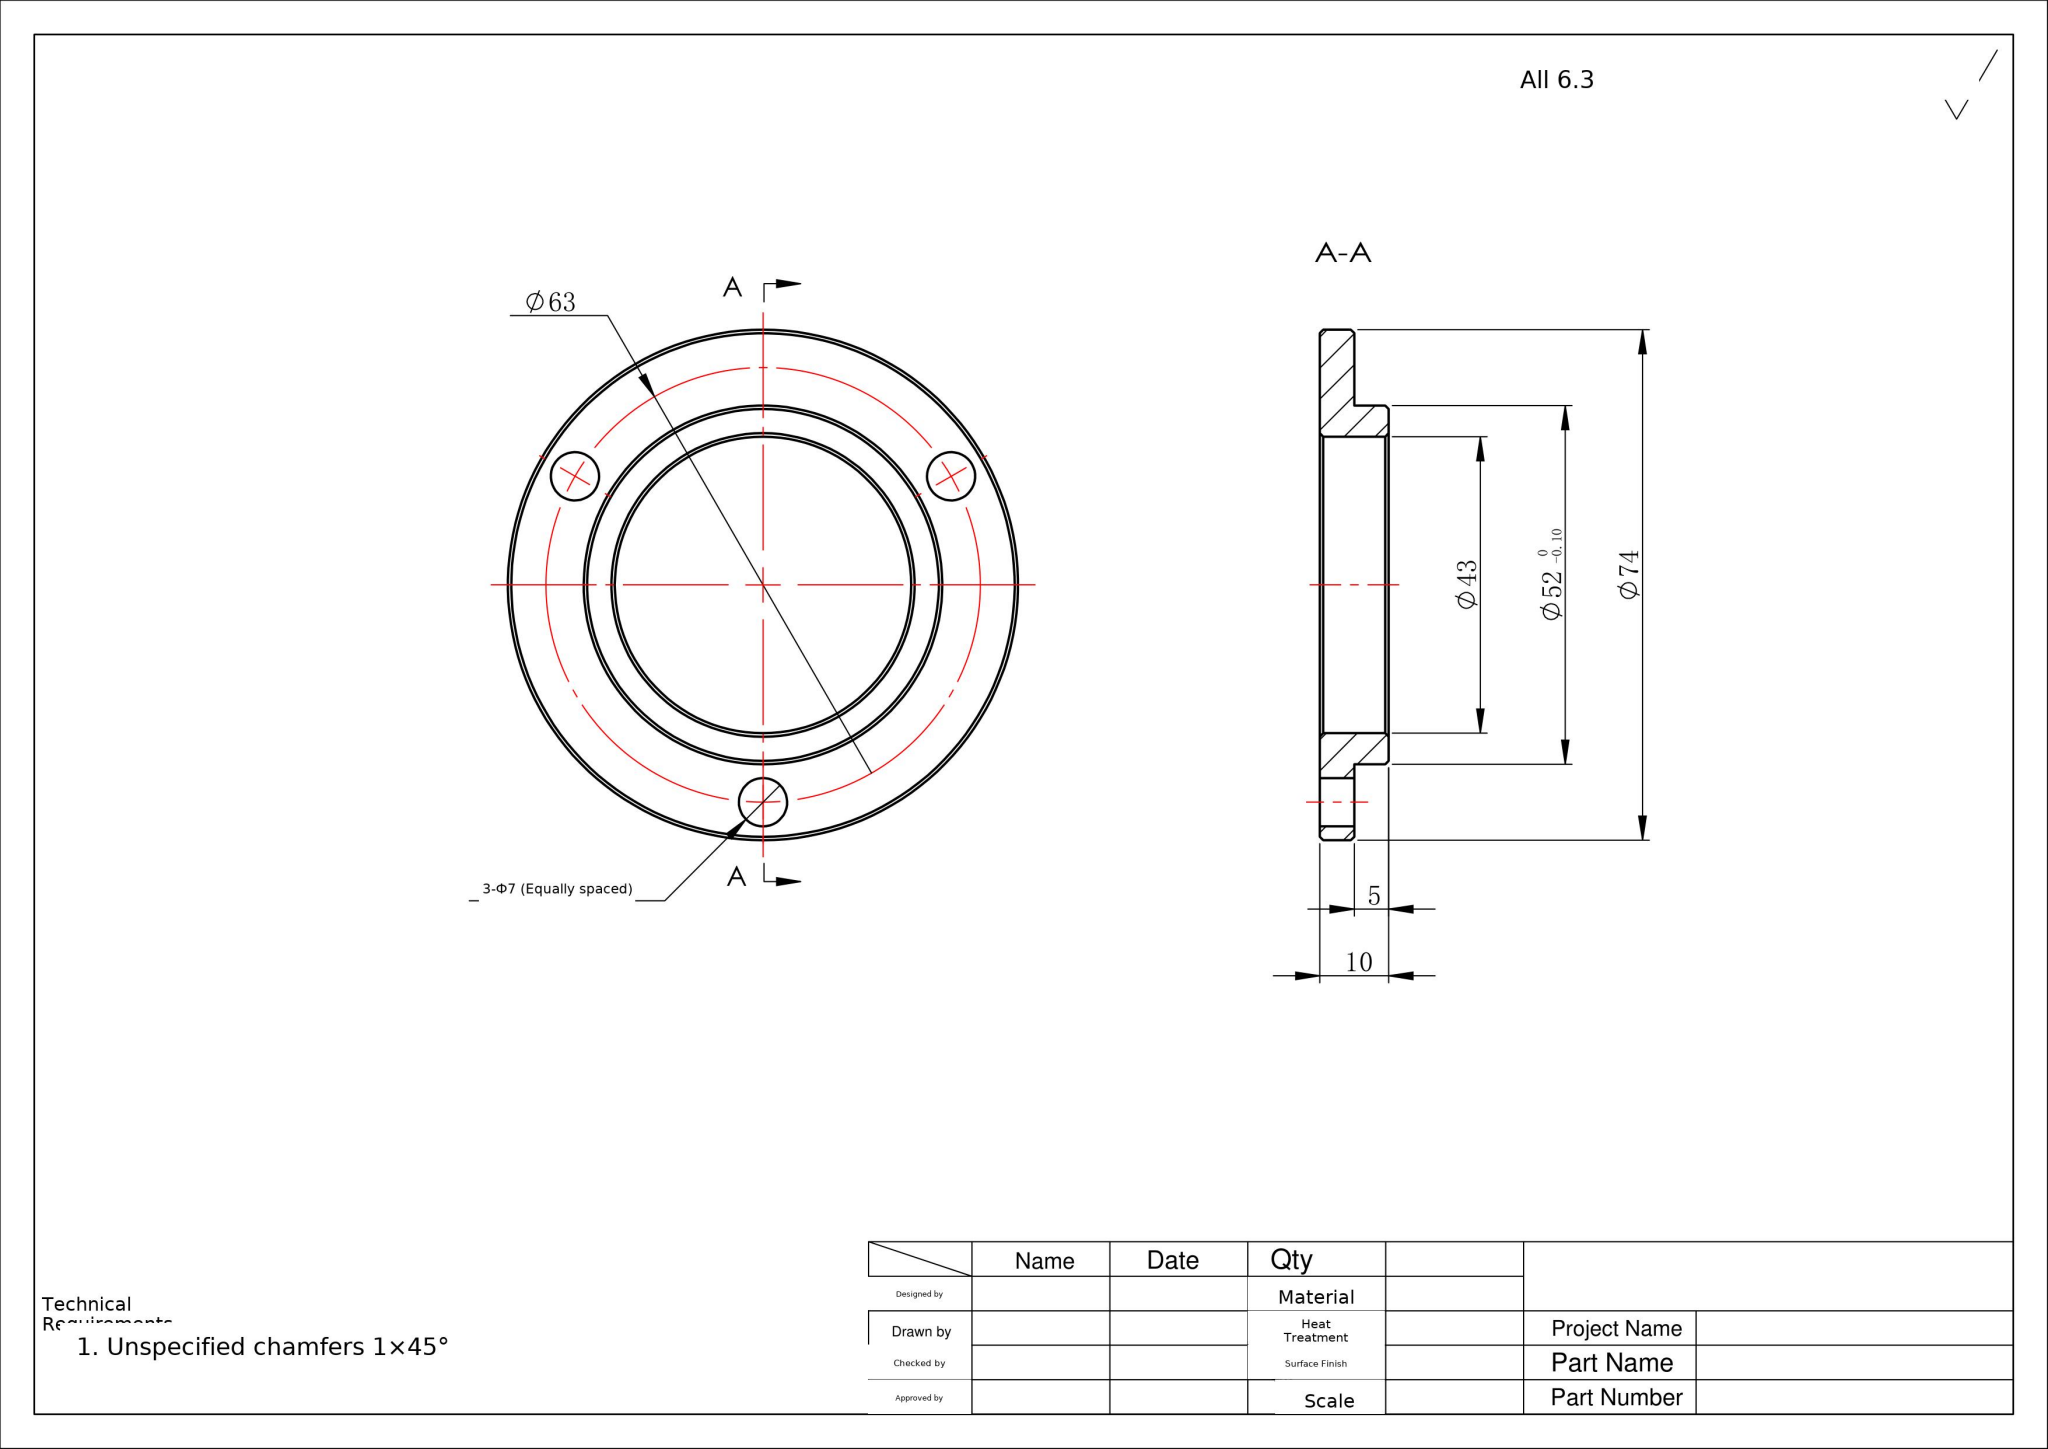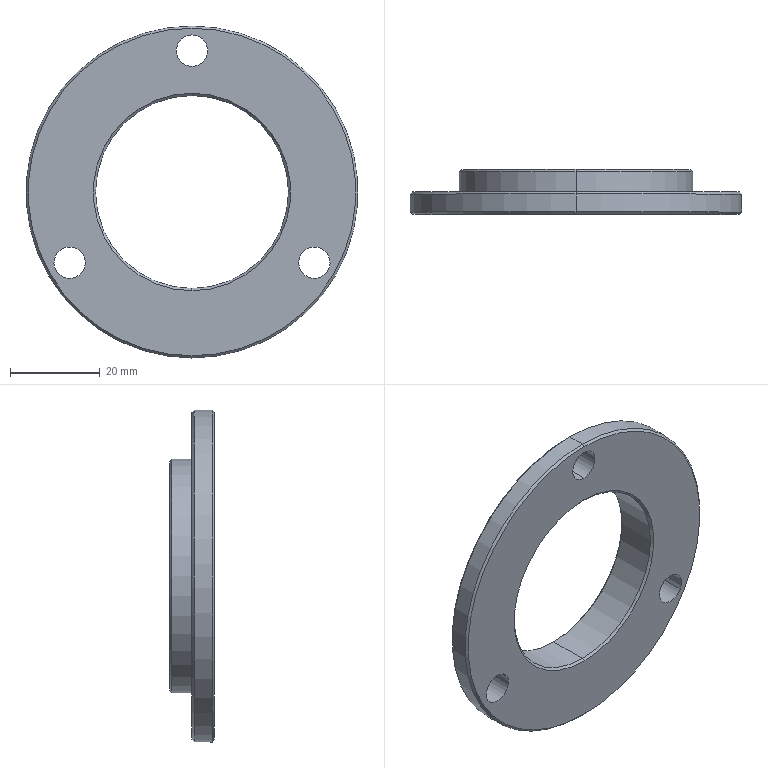Part | SolidWorks | mm | 1 solid | 25 faces | box 74 x 10 x 74 mm | volume 16911 mm3 | cylinder 12 | cone 10 | plane 3 | commonest cylinder face diameters 7 x6 43 x2 52 x2 74 x2
build123d program:
from build123d import *

# Parameters (mm, degrees)
SKETCH2_R          = 3.5
CUT_EXTRUDE1_DEPTH = 54.273
CIRPATTERN1_COUNT  = 3
CHAMFER1_SIZE      = 0.5


with BuildPart() as part:
    # Sketch1 → Revolve1 (revolve)
    with BuildSketch(Plane.XY, mode=Mode.PRIVATE) as revolve1_sk:
        Polygon((21.5, 0), (37, 0), (37, 5), (26, 5), (26, 10), (21.5, 10), align=None)
    revolve(revolve1_sk.sketch.rotate(Axis((0, 0, 0), (0, 1, 0)), 90), axis=Axis((0, 0, 0), (0, 1, 0)))

    # Sketch2 → Cut-Extrude1 (cut, through all)
    with BuildSketch(Plane.XZ):
        with Locations(Location((0, 31.5, 0), (0, 0, 270))):
            Circle(SKETCH2_R)
    cut_extrude1 = extrude(amount=-CUT_EXTRUDE1_DEPTH, mode=Mode.SUBTRACT)

    # CirPattern1: Cut-Extrude1 ×3 about axis
    cirpattern1_axis = Axis((0, 0, 0), (0, 1, 0))
    for i in range(1, CIRPATTERN1_COUNT):
        add(cut_extrude1.rotate(cirpattern1_axis, i * 360 / CIRPATTERN1_COUNT), mode=Mode.SUBTRACT)

    # Chamfer1
    chamfer1_edges = [part.edges().sort_by_distance(p)[0] for p in [
        (0, 0, 37),
        (0, 0, 21.5),
        (0, 10, 21.5),
        (0, 10, 26),
        (0, 5, 37),
    ]]
    chamfer(chamfer1_edges, length=CHAMFER1_SIZE)


solid = part.part
STEP:
#1=CARTESIAN_POINT('',(0.,5.,36.5));
#2=VERTEX_POINT('',#1);
#3=CARTESIAN_POINT('',(-0.,5.,-36.5));
#4=VERTEX_POINT('',#3);
#5=CARTESIAN_POINT('',(0.,5.,-0.));
#6=DIRECTION('',(-0.,1.,0.));
#7=DIRECTION('',(0.,0.,1.));
#8=AXIS2_PLACEMENT_3D('',#5,#6,#7);
#9=CIRCLE('',#8,36.5);
#10=EDGE_CURVE('',#2,#4,#9,.T.);
#11=ORIENTED_EDGE('',*,*,#10,.F.);
#12=CARTESIAN_POINT('',(0.,4.5,37.));
#13=VERTEX_POINT('',#12);
#14=CARTESIAN_POINT('',(0.,4.5,37.));
#15=DIRECTION('',(0.,-0.7071,0.7071));
#16=VECTOR('',#15,1000.);
#17=LINE('',#14,#16);
#18=EDGE_CURVE('',#2,#13,#17,.T.);
#19=ORIENTED_EDGE('',*,*,#18,.T.);
#20=CARTESIAN_POINT('',(-0.,4.5,-37.));
#21=VERTEX_POINT('',#20);
#22=CARTESIAN_POINT('',(0.,4.5,-0.));
#23=DIRECTION('',(0.,-1.,-0.));
#24=DIRECTION('',(0.,0.,1.));
#25=AXIS2_PLACEMENT_3D('',#22,#23,#24);
#26=CIRCLE('',#25,37.);
#27=EDGE_CURVE('',#21,#13,#26,.T.);
#28=ORIENTED_EDGE('',*,*,#27,.F.);
#29=CARTESIAN_POINT('',(-0.,4.5,-37.));
#30=DIRECTION('',(-0.,-0.7071,-0.7071));
#31=VECTOR('',#30,1000.);
#32=LINE('',#29,#31);
#33=EDGE_CURVE('',#4,#21,#32,.T.);
#34=ORIENTED_EDGE('',*,*,#33,.F.);
#35=EDGE_LOOP('',(#11,#19,#28,#34));
#36=FACE_OUTER_BOUND('',#35,.T.);
#37=CARTESIAN_POINT('',(0.,4.5,-0.));
#38=DIRECTION('',(0.,-1.,-0.));
#39=DIRECTION('',(-0.,0.,-1.));
#40=AXIS2_PLACEMENT_3D('',#37,#38,#39);
#41=CONICAL_SURFACE('',#40,37.,0.7854);
#42=ADVANCED_FACE('',(#36),#41,.T.);
#43=CARTESIAN_POINT('',(0.,0.,-36.5));
#44=VERTEX_POINT('',#43);
#45=CARTESIAN_POINT('',(0.,-0.,36.5));
#46=VERTEX_POINT('',#45);
#47=CARTESIAN_POINT('',(0.,0.,-0.));
#48=DIRECTION('',(0.,-1.,-0.));
#49=DIRECTION('',(-0.,-0.,-1.));
#50=AXIS2_PLACEMENT_3D('',#47,#48,#49);
#51=CIRCLE('',#50,36.5);
#52=EDGE_CURVE('',#44,#46,#51,.T.);
#53=ORIENTED_EDGE('',*,*,#52,.F.);
#54=CARTESIAN_POINT('',(-0.,0.5,-37.));
#55=VERTEX_POINT('',#54);
#56=CARTESIAN_POINT('',(0.,-0.,-36.5));
#57=DIRECTION('',(0.,0.7071,-0.7071));
#58=VECTOR('',#57,1000.);
#59=LINE('',#56,#58);
#60=EDGE_CURVE('',#44,#55,#59,.T.);
#61=ORIENTED_EDGE('',*,*,#60,.T.);
#62=CARTESIAN_POINT('',(0.,0.5,37.));
#63=VERTEX_POINT('',#62);
#64=CARTESIAN_POINT('',(0.,0.5,-0.));
#65=DIRECTION('',(-0.,1.,0.));
#66=DIRECTION('',(-0.,0.,-1.));
#67=AXIS2_PLACEMENT_3D('',#64,#65,#66);
#68=CIRCLE('',#67,37.);
#69=EDGE_CURVE('',#63,#55,#68,.T.);
#70=ORIENTED_EDGE('',*,*,#69,.F.);
#71=CARTESIAN_POINT('',(0.,0.,36.5));
#72=DIRECTION('',(0.,0.7071,0.7071));
#73=VECTOR('',#72,1000.);
#74=LINE('',#71,#73);
#75=EDGE_CURVE('',#46,#63,#74,.T.);
#76=ORIENTED_EDGE('',*,*,#75,.F.);
#77=EDGE_LOOP('',(#53,#61,#70,#76));
#78=FACE_OUTER_BOUND('',#77,.T.);
#79=CARTESIAN_POINT('',(0.,0.,-0.));
#80=DIRECTION('',(-0.,1.,0.));
#81=DIRECTION('',(0.,0.,1.));
#82=AXIS2_PLACEMENT_3D('',#79,#80,#81);
#83=CONICAL_SURFACE('',#82,36.5,0.7854);
#84=ADVANCED_FACE('',(#78),#83,.T.);
#85=CARTESIAN_POINT('',(0.,0.5,21.5));
#86=VERTEX_POINT('',#85);
#87=CARTESIAN_POINT('',(-0.,0.5,-21.5));
#88=VERTEX_POINT('',#87);
#89=CARTESIAN_POINT('',(0.,0.5,-0.));
#90=DIRECTION('',(0.,-1.,-0.));
#91=DIRECTION('',(-0.,0.,-1.));
#92=AXIS2_PLACEMENT_3D('',#89,#90,#91);
#93=CIRCLE('',#92,21.5);
#94=EDGE_CURVE('',#86,#88,#93,.T.);
#95=ORIENTED_EDGE('',*,*,#94,.F.);
#96=CARTESIAN_POINT('',(0.,0.,22.));
#97=VERTEX_POINT('',#96);
#98=CARTESIAN_POINT('',(0.,0.5,21.5));
#99=DIRECTION('',(0.,-0.7071,0.7071));
#100=VECTOR('',#99,1000.);
#101=LINE('',#98,#100);
#102=EDGE_CURVE('',#86,#97,#101,.T.);
#103=ORIENTED_EDGE('',*,*,#102,.T.);
#104=CARTESIAN_POINT('',(-0.,0.,-22.));
#105=VERTEX_POINT('',#104);
#106=CARTESIAN_POINT('',(0.,0.,-0.));
#107=DIRECTION('',(-0.,1.,0.));
#108=DIRECTION('',(-0.,-0.,-1.));
#109=AXIS2_PLACEMENT_3D('',#106,#107,#108);
#110=CIRCLE('',#109,22.);
#111=EDGE_CURVE('',#105,#97,#110,.T.);
#112=ORIENTED_EDGE('',*,*,#111,.F.);
#113=CARTESIAN_POINT('',(-0.,0.5,-21.5));
#114=DIRECTION('',(-0.,-0.7071,-0.7071));
#115=VECTOR('',#114,1000.);
#116=LINE('',#113,#115);
#117=EDGE_CURVE('',#88,#105,#116,.T.);
#118=ORIENTED_EDGE('',*,*,#117,.F.);
#119=EDGE_LOOP('',(#95,#103,#112,#118));
#120=FACE_OUTER_BOUND('',#119,.T.);
#121=CARTESIAN_POINT('',(0.,0.5,-0.));
#122=DIRECTION('',(0.,-1.,-0.));
#123=DIRECTION('',(-0.,0.,-1.));
#124=AXIS2_PLACEMENT_3D('',#121,#122,#123);
#125=CONICAL_SURFACE('',#124,21.5,0.7854);
#126=ADVANCED_FACE('',(#120),#125,.F.);
#127=CARTESIAN_POINT('',(0.,10.,25.5));
#128=VERTEX_POINT('',#127);
#129=CARTESIAN_POINT('',(-0.,10.,-25.5));
#130=VERTEX_POINT('',#129);
#131=CARTESIAN_POINT('',(0.,10.,-0.));
#132=DIRECTION('',(-0.,1.,0.));
#133=DIRECTION('',(0.,0.,1.));
#134=AXIS2_PLACEMENT_3D('',#131,#132,#133);
#135=CIRCLE('',#134,25.5);
#136=EDGE_CURVE('',#128,#130,#135,.T.);
#137=ORIENTED_EDGE('',*,*,#136,.F.);
#138=CARTESIAN_POINT('',(0.,9.5,26.));
#139=VERTEX_POINT('',#138);
#140=CARTESIAN_POINT('',(0.,9.5,26.));
#141=DIRECTION('',(0.,-0.7071,0.7071));
#142=VECTOR('',#141,1000.);
#143=LINE('',#140,#142);
#144=EDGE_CURVE('',#128,#139,#143,.T.);
#145=ORIENTED_EDGE('',*,*,#144,.T.);
#146=CARTESIAN_POINT('',(-0.,9.5,-26.));
#147=VERTEX_POINT('',#146);
#148=CARTESIAN_POINT('',(0.,9.5,-0.));
#149=DIRECTION('',(0.,-1.,-0.));
#150=DIRECTION('',(0.,0.,1.));
#151=AXIS2_PLACEMENT_3D('',#148,#149,#150);
#152=CIRCLE('',#151,26.);
#153=EDGE_CURVE('',#147,#139,#152,.T.);
#154=ORIENTED_EDGE('',*,*,#153,.F.);
#155=CARTESIAN_POINT('',(-0.,9.5,-26.));
#156=DIRECTION('',(-0.,-0.7071,-0.7071));
#157=VECTOR('',#156,1000.);
#158=LINE('',#155,#157);
#159=EDGE_CURVE('',#130,#147,#158,.T.);
#160=ORIENTED_EDGE('',*,*,#159,.F.);
#161=EDGE_LOOP('',(#137,#145,#154,#160));
#162=FACE_OUTER_BOUND('',#161,.T.);
#163=CARTESIAN_POINT('',(0.,9.5,-0.));
#164=DIRECTION('',(0.,-1.,-0.));
#165=DIRECTION('',(-0.,0.,-1.));
#166=AXIS2_PLACEMENT_3D('',#163,#164,#165);
#167=CONICAL_SURFACE('',#166,26.,0.7854);
#168=ADVANCED_FACE('',(#162),#167,.T.);
#169=CARTESIAN_POINT('',(-0.,9.5,-21.5));
#170=VERTEX_POINT('',#169);
#171=CARTESIAN_POINT('',(0.,9.5,21.5));
#172=VERTEX_POINT('',#171);
#173=CARTESIAN_POINT('',(0.,9.5,-0.));
#174=DIRECTION('',(-0.,1.,0.));
#175=DIRECTION('',(0.,0.,1.));
#176=AXIS2_PLACEMENT_3D('',#173,#174,#175);
#177=CIRCLE('',#176,21.5);
#178=EDGE_CURVE('',#170,#172,#177,.T.);
#179=ORIENTED_EDGE('',*,*,#178,.F.);
#180=CARTESIAN_POINT('',(0.,10.,-22.));
#181=VERTEX_POINT('',#180);
#182=CARTESIAN_POINT('',(0.,10.,-22.));
#183=DIRECTION('',(0.,0.7071,-0.7071));
#184=VECTOR('',#183,1000.);
#185=LINE('',#182,#184);
#186=EDGE_CURVE('',#170,#181,#185,.T.);
#187=ORIENTED_EDGE('',*,*,#186,.T.);
#188=CARTESIAN_POINT('',(0.,10.,22.));
#189=VERTEX_POINT('',#188);
#190=CARTESIAN_POINT('',(0.,10.,-0.));
#191=DIRECTION('',(0.,-1.,-0.));
#192=DIRECTION('',(0.,0.,1.));
#193=AXIS2_PLACEMENT_3D('',#190,#191,#192);
#194=CIRCLE('',#193,22.);
#195=EDGE_CURVE('',#189,#181,#194,.T.);
#196=ORIENTED_EDGE('',*,*,#195,.F.);
#197=CARTESIAN_POINT('',(0.,10.,22.));
#198=DIRECTION('',(0.,0.7071,0.7071));
#199=VECTOR('',#198,1000.);
#200=LINE('',#197,#199);
#201=EDGE_CURVE('',#172,#189,#200,.T.);
#202=ORIENTED_EDGE('',*,*,#201,.F.);
#203=EDGE_LOOP('',(#179,#187,#196,#202));
#204=FACE_OUTER_BOUND('',#203,.T.);
#205=CARTESIAN_POINT('',(0.,10.,-0.));
#206=DIRECTION('',(-0.,1.,0.));
#207=DIRECTION('',(0.,0.,1.));
#208=AXIS2_PLACEMENT_3D('',#205,#206,#207);
#209=CONICAL_SURFACE('',#208,22.,0.7854);
#210=ADVANCED_FACE('',(#204),#209,.F.);
#211=CARTESIAN_POINT('',(-24.249,5.,-14.));
#212=VERTEX_POINT('',#211);
#213=CARTESIAN_POINT('',(-30.311,5.,-17.5));
#214=VERTEX_POINT('',#213);
#215=CARTESIAN_POINT('',(-27.28,5.,-15.75));
#216=DIRECTION('',(-0.,1.,0.));
#217=DIRECTION('',(-0.866,0.,-0.5));
#218=AXIS2_PLACEMENT_3D('',#215,#216,#217);
#219=CIRCLE('',#218,3.5);
#220=EDGE_CURVE('',#212,#214,#219,.T.);
#221=ORIENTED_EDGE('',*,*,#220,.T.);
#222=CARTESIAN_POINT('',(-30.311,0.,-17.5));
#223=VERTEX_POINT('',#222);
#224=CARTESIAN_POINT('',(-30.311,10.,-17.5));
#225=DIRECTION('',(0.,-1.,-0.));
#226=VECTOR('',#225,1000.);
#227=LINE('',#224,#226);
#228=EDGE_CURVE('',#214,#223,#227,.T.);
#229=ORIENTED_EDGE('',*,*,#228,.T.);
#230=CARTESIAN_POINT('',(-24.249,0.,-14.));
#231=VERTEX_POINT('',#230);
#232=CARTESIAN_POINT('',(-27.28,0.,-15.75));
#233=DIRECTION('',(0.,-1.,-0.));
#234=DIRECTION('',(0.866,0.,0.5));
#235=AXIS2_PLACEMENT_3D('',#232,#233,#234);
#236=CIRCLE('',#235,3.5);
#237=EDGE_CURVE('',#223,#231,#236,.T.);
#238=ORIENTED_EDGE('',*,*,#237,.T.);
#239=CARTESIAN_POINT('',(-24.249,10.,-14.));
#240=DIRECTION('',(0.,-1.,-0.));
#241=VECTOR('',#240,1000.);
#242=LINE('',#239,#241);
#243=EDGE_CURVE('',#212,#231,#242,.T.);
#244=ORIENTED_EDGE('',*,*,#243,.F.);
#245=EDGE_LOOP('',(#221,#229,#238,#244));
#246=FACE_OUTER_BOUND('',#245,.T.);
#247=CARTESIAN_POINT('',(-27.28,10.,-15.75));
#248=DIRECTION('',(0.,-1.,-0.));
#249=DIRECTION('',(0.866,0.,0.5));
#250=AXIS2_PLACEMENT_3D('',#247,#248,#249);
#251=CYLINDRICAL_SURFACE('',#250,3.5);
#252=ADVANCED_FACE('',(#246),#251,.F.);
#253=CARTESIAN_POINT('',(24.249,5.,-14.));
#254=VERTEX_POINT('',#253);
#255=CARTESIAN_POINT('',(30.311,5.,-17.5));
#256=VERTEX_POINT('',#255);
#257=CARTESIAN_POINT('',(27.28,5.,-15.75));
#258=DIRECTION('',(-0.,1.,0.));
#259=DIRECTION('',(0.866,0.,-0.5));
#260=AXIS2_PLACEMENT_3D('',#257,#258,#259);
#261=CIRCLE('',#260,3.5);
#262=EDGE_CURVE('',#254,#256,#261,.T.);
#263=ORIENTED_EDGE('',*,*,#262,.T.);
#264=CARTESIAN_POINT('',(30.311,0.,-17.5));
#265=VERTEX_POINT('',#264);
#266=CARTESIAN_POINT('',(30.311,10.,-17.5));
#267=DIRECTION('',(0.,-1.,-0.));
#268=VECTOR('',#267,1000.);
#269=LINE('',#266,#268);
#270=EDGE_CURVE('',#256,#265,#269,.T.);
#271=ORIENTED_EDGE('',*,*,#270,.T.);
#272=CARTESIAN_POINT('',(24.249,0.,-14.));
#273=VERTEX_POINT('',#272);
#274=CARTESIAN_POINT('',(27.28,0.,-15.75));
#275=DIRECTION('',(0.,-1.,-0.));
#276=DIRECTION('',(-0.866,0.,0.5));
#277=AXIS2_PLACEMENT_3D('',#274,#275,#276);
#278=CIRCLE('',#277,3.5);
#279=EDGE_CURVE('',#265,#273,#278,.T.);
#280=ORIENTED_EDGE('',*,*,#279,.T.);
#281=CARTESIAN_POINT('',(24.249,10.,-14.));
#282=DIRECTION('',(0.,-1.,-0.));
#283=VECTOR('',#282,1000.);
#284=LINE('',#281,#283);
#285=EDGE_CURVE('',#254,#273,#284,.T.);
#286=ORIENTED_EDGE('',*,*,#285,.F.);
#287=EDGE_LOOP('',(#263,#271,#280,#286));
#288=FACE_OUTER_BOUND('',#287,.T.);
#289=CARTESIAN_POINT('',(27.28,10.,-15.75));
#290=DIRECTION('',(0.,-1.,-0.));
#291=DIRECTION('',(-0.866,0.,0.5));
#292=AXIS2_PLACEMENT_3D('',#289,#290,#291);
#293=CYLINDRICAL_SURFACE('',#292,3.5);
#294=ADVANCED_FACE('',(#288),#293,.F.);
#295=CARTESIAN_POINT('',(-0.,5.,28.));
#296=VERTEX_POINT('',#295);
#297=CARTESIAN_POINT('',(-0.,5.,35.));
#298=VERTEX_POINT('',#297);
#299=CARTESIAN_POINT('',(-0.,5.,31.5));
#300=DIRECTION('',(-0.,1.,0.));
#301=DIRECTION('',(0.,0.,1.));
#302=AXIS2_PLACEMENT_3D('',#299,#300,#301);
#303=CIRCLE('',#302,3.5);
#304=EDGE_CURVE('',#296,#298,#303,.T.);
#305=ORIENTED_EDGE('',*,*,#304,.T.);
#306=CARTESIAN_POINT('',(-0.,-0.,35.));
#307=VERTEX_POINT('',#306);
#308=CARTESIAN_POINT('',(-0.,10.,35.));
#309=DIRECTION('',(0.,-1.,-0.));
#310=VECTOR('',#309,1000.);
#311=LINE('',#308,#310);
#312=EDGE_CURVE('',#298,#307,#311,.T.);
#313=ORIENTED_EDGE('',*,*,#312,.T.);
#314=CARTESIAN_POINT('',(-0.,-0.,28.));
#315=VERTEX_POINT('',#314);
#316=CARTESIAN_POINT('',(-0.,-0.,31.5));
#317=DIRECTION('',(0.,-1.,-0.));
#318=DIRECTION('',(-0.,0.,-1.));
#319=AXIS2_PLACEMENT_3D('',#316,#317,#318);
#320=CIRCLE('',#319,3.5);
#321=EDGE_CURVE('',#307,#315,#320,.T.);
#322=ORIENTED_EDGE('',*,*,#321,.T.);
#323=CARTESIAN_POINT('',(-0.,10.,28.));
#324=DIRECTION('',(0.,-1.,-0.));
#325=VECTOR('',#324,1000.);
#326=LINE('',#323,#325);
#327=EDGE_CURVE('',#296,#315,#326,.T.);
#328=ORIENTED_EDGE('',*,*,#327,.F.);
#329=EDGE_LOOP('',(#305,#313,#322,#328));
#330=FACE_OUTER_BOUND('',#329,.T.);
#331=CARTESIAN_POINT('',(-0.,10.,31.5));
#332=DIRECTION('',(0.,-1.,-0.));
#333=DIRECTION('',(-0.,0.,-1.));
#334=AXIS2_PLACEMENT_3D('',#331,#332,#333);
#335=CYLINDRICAL_SURFACE('',#334,3.5);
#336=ADVANCED_FACE('',(#330),#335,.F.);
#337=ORIENTED_EDGE('',*,*,#178,.T.);
#338=CARTESIAN_POINT('',(0.,0.,21.5));
#339=DIRECTION('',(0.,-1.,-0.));
#340=VECTOR('',#339,1000.);
#341=LINE('',#338,#340);
#342=EDGE_CURVE('',#172,#86,#341,.T.);
#343=ORIENTED_EDGE('',*,*,#342,.T.);
#344=ORIENTED_EDGE('',*,*,#94,.T.);
#345=CARTESIAN_POINT('',(-0.,-0.,-21.5));
#346=DIRECTION('',(0.,-1.,-0.));
#347=VECTOR('',#346,1000.);
#348=LINE('',#345,#347);
#349=EDGE_CURVE('',#170,#88,#348,.T.);
#350=ORIENTED_EDGE('',*,*,#349,.F.);
#351=EDGE_LOOP('',(#337,#343,#344,#350));
#352=FACE_OUTER_BOUND('',#351,.T.);
#353=CARTESIAN_POINT('',(0.,0.,-0.));
#354=DIRECTION('',(0.,-1.,-0.));
#355=DIRECTION('',(-0.,-0.,-1.));
#356=AXIS2_PLACEMENT_3D('',#353,#354,#355);
#357=CYLINDRICAL_SURFACE('',#356,21.5);
#358=ADVANCED_FACE('',(#352),#357,.F.);
#359=ORIENTED_EDGE('',*,*,#153,.T.);
#360=CARTESIAN_POINT('',(0.,5.,26.));
#361=VERTEX_POINT('',#360);
#362=CARTESIAN_POINT('',(0.,0.,26.));
#363=DIRECTION('',(0.,-1.,-0.));
#364=VECTOR('',#363,1000.);
#365=LINE('',#362,#364);
#366=EDGE_CURVE('',#139,#361,#365,.T.);
#367=ORIENTED_EDGE('',*,*,#366,.T.);
#368=CARTESIAN_POINT('',(-0.,5.,-26.));
#369=VERTEX_POINT('',#368);
#370=CARTESIAN_POINT('',(0.,5.,-0.));
#371=DIRECTION('',(0.,-1.,-0.));
#372=DIRECTION('',(-0.,0.,-1.));
#373=AXIS2_PLACEMENT_3D('',#370,#371,#372);
#374=CIRCLE('',#373,26.);
#375=EDGE_CURVE('',#369,#361,#374,.T.);
#376=ORIENTED_EDGE('',*,*,#375,.F.);
#377=CARTESIAN_POINT('',(-0.,-0.,-26.));
#378=DIRECTION('',(0.,-1.,-0.));
#379=VECTOR('',#378,1000.);
#380=LINE('',#377,#379);
#381=EDGE_CURVE('',#147,#369,#380,.T.);
#382=ORIENTED_EDGE('',*,*,#381,.F.);
#383=EDGE_LOOP('',(#359,#367,#376,#382));
#384=FACE_OUTER_BOUND('',#383,.T.);
#385=CARTESIAN_POINT('',(0.,0.,-0.));
#386=DIRECTION('',(0.,-1.,-0.));
#387=DIRECTION('',(-0.,-0.,-1.));
#388=AXIS2_PLACEMENT_3D('',#385,#386,#387);
#389=CYLINDRICAL_SURFACE('',#388,26.);
#390=ADVANCED_FACE('',(#384),#389,.T.);
#391=ORIENTED_EDGE('',*,*,#27,.T.);
#392=CARTESIAN_POINT('',(0.,0.,37.));
#393=DIRECTION('',(0.,-1.,-0.));
#394=VECTOR('',#393,1000.);
#395=LINE('',#392,#394);
#396=EDGE_CURVE('',#13,#63,#395,.T.);
#397=ORIENTED_EDGE('',*,*,#396,.T.);
#398=ORIENTED_EDGE('',*,*,#69,.T.);
#399=CARTESIAN_POINT('',(-0.,-0.,-37.));
#400=DIRECTION('',(0.,-1.,-0.));
#401=VECTOR('',#400,1000.);
#402=LINE('',#399,#401);
#403=EDGE_CURVE('',#21,#55,#402,.T.);
#404=ORIENTED_EDGE('',*,*,#403,.F.);
#405=EDGE_LOOP('',(#391,#397,#398,#404));
#406=FACE_OUTER_BOUND('',#405,.T.);
#407=CARTESIAN_POINT('',(0.,0.,-0.));
#408=DIRECTION('',(0.,-1.,-0.));
#409=DIRECTION('',(-0.,-0.,-1.));
#410=AXIS2_PLACEMENT_3D('',#407,#408,#409);
#411=CYLINDRICAL_SURFACE('',#410,37.);
#412=ADVANCED_FACE('',(#406),#411,.T.);
#413=ORIENTED_EDGE('',*,*,#396,.F.);
#414=CARTESIAN_POINT('',(0.,4.5,-0.));
#415=DIRECTION('',(0.,-1.,-0.));
#416=DIRECTION('',(0.,0.,1.));
#417=AXIS2_PLACEMENT_3D('',#414,#415,#416);
#418=CIRCLE('',#417,37.);
#419=EDGE_CURVE('',#13,#21,#418,.T.);
#420=ORIENTED_EDGE('',*,*,#419,.T.);
#421=ORIENTED_EDGE('',*,*,#403,.T.);
#422=CARTESIAN_POINT('',(0.,0.5,-0.));
#423=DIRECTION('',(-0.,1.,0.));
#424=DIRECTION('',(-0.,0.,-1.));
#425=AXIS2_PLACEMENT_3D('',#422,#423,#424);
#426=CIRCLE('',#425,37.);
#427=EDGE_CURVE('',#55,#63,#426,.T.);
#428=ORIENTED_EDGE('',*,*,#427,.T.);
#429=EDGE_LOOP('',(#413,#420,#421,#428));
#430=FACE_OUTER_BOUND('',#429,.T.);
#431=CARTESIAN_POINT('',(0.,0.,-0.));
#432=DIRECTION('',(0.,-1.,-0.));
#433=DIRECTION('',(-0.,-0.,-1.));
#434=AXIS2_PLACEMENT_3D('',#431,#432,#433);
#435=CYLINDRICAL_SURFACE('',#434,37.);
#436=ADVANCED_FACE('',(#430),#435,.T.);
#437=CARTESIAN_POINT('',(0.,5.,-0.));
#438=DIRECTION('',(-0.,1.,0.));
#439=DIRECTION('',(0.,0.,1.));
#440=AXIS2_PLACEMENT_3D('',#437,#438,#439);
#441=CIRCLE('',#440,36.5);
#442=EDGE_CURVE('',#4,#2,#441,.T.);
#443=ORIENTED_EDGE('',*,*,#442,.T.);
#444=ORIENTED_EDGE('',*,*,#10,.T.);
#445=EDGE_LOOP('',(#443,#444));
#446=FACE_OUTER_BOUND('',#445,.T.);
#447=ORIENTED_EDGE('',*,*,#220,.F.);
#448=CARTESIAN_POINT('',(-27.28,5.,-15.75));
#449=DIRECTION('',(-0.,1.,0.));
#450=DIRECTION('',(-0.866,0.,-0.5));
#451=AXIS2_PLACEMENT_3D('',#448,#449,#450);
#452=CIRCLE('',#451,3.5);
#453=EDGE_CURVE('',#214,#212,#452,.T.);
#454=ORIENTED_EDGE('',*,*,#453,.F.);
#455=EDGE_LOOP('',(#447,#454));
#456=FACE_BOUND('',#455,.T.);
#457=ORIENTED_EDGE('',*,*,#262,.F.);
#458=CARTESIAN_POINT('',(27.28,5.,-15.75));
#459=DIRECTION('',(-0.,1.,0.));
#460=DIRECTION('',(0.866,0.,-0.5));
#461=AXIS2_PLACEMENT_3D('',#458,#459,#460);
#462=CIRCLE('',#461,3.5);
#463=EDGE_CURVE('',#256,#254,#462,.T.);
#464=ORIENTED_EDGE('',*,*,#463,.F.);
#465=EDGE_LOOP('',(#457,#464));
#466=FACE_BOUND('',#465,.T.);
#467=ORIENTED_EDGE('',*,*,#304,.F.);
#468=CARTESIAN_POINT('',(-0.,5.,31.5));
#469=DIRECTION('',(-0.,1.,0.));
#470=DIRECTION('',(0.,0.,1.));
#471=AXIS2_PLACEMENT_3D('',#468,#469,#470);
#472=CIRCLE('',#471,3.5);
#473=EDGE_CURVE('',#298,#296,#472,.T.);
#474=ORIENTED_EDGE('',*,*,#473,.F.);
#475=EDGE_LOOP('',(#467,#474));
#476=FACE_BOUND('',#475,.T.);
#477=ORIENTED_EDGE('',*,*,#375,.T.);
#478=CARTESIAN_POINT('',(0.,5.,-0.));
#479=DIRECTION('',(0.,-1.,-0.));
#480=DIRECTION('',(-0.,0.,-1.));
#481=AXIS2_PLACEMENT_3D('',#478,#479,#480);
#482=CIRCLE('',#481,26.);
#483=EDGE_CURVE('',#361,#369,#482,.T.);
#484=ORIENTED_EDGE('',*,*,#483,.T.);
#485=EDGE_LOOP('',(#477,#484));
#486=FACE_BOUND('',#485,.T.);
#487=CARTESIAN_POINT('',(37.,5.,0.));
#488=DIRECTION('',(-0.,1.,-0.));
#489=DIRECTION('',(0.,0.,1.));
#490=AXIS2_PLACEMENT_3D('',#487,#488,#489);
#491=PLANE('',#490);
#492=ADVANCED_FACE('',(#446,#456,#466,#476,#486),#491,.T.);
#493=ORIENTED_EDGE('',*,*,#366,.F.);
#494=CARTESIAN_POINT('',(0.,9.5,-0.));
#495=DIRECTION('',(0.,-1.,-0.));
#496=DIRECTION('',(0.,0.,1.));
#497=AXIS2_PLACEMENT_3D('',#494,#495,#496);
#498=CIRCLE('',#497,26.);
#499=EDGE_CURVE('',#139,#147,#498,.T.);
#500=ORIENTED_EDGE('',*,*,#499,.T.);
#501=ORIENTED_EDGE('',*,*,#381,.T.);
#502=ORIENTED_EDGE('',*,*,#483,.F.);
#503=EDGE_LOOP('',(#493,#500,#501,#502));
#504=FACE_OUTER_BOUND('',#503,.T.);
#505=CARTESIAN_POINT('',(0.,0.,-0.));
#506=DIRECTION('',(0.,-1.,-0.));
#507=DIRECTION('',(-0.,-0.,-1.));
#508=AXIS2_PLACEMENT_3D('',#505,#506,#507);
#509=CYLINDRICAL_SURFACE('',#508,26.);
#510=ADVANCED_FACE('',(#504),#509,.T.);
#511=ORIENTED_EDGE('',*,*,#195,.T.);
#512=CARTESIAN_POINT('',(0.,10.,-0.));
#513=DIRECTION('',(0.,-1.,-0.));
#514=DIRECTION('',(0.,0.,1.));
#515=AXIS2_PLACEMENT_3D('',#512,#513,#514);
#516=CIRCLE('',#515,22.);
#517=EDGE_CURVE('',#181,#189,#516,.T.);
#518=ORIENTED_EDGE('',*,*,#517,.T.);
#519=EDGE_LOOP('',(#511,#518));
#520=FACE_BOUND('',#519,.T.);
#521=CARTESIAN_POINT('',(0.,10.,-0.));
#522=DIRECTION('',(-0.,1.,0.));
#523=DIRECTION('',(0.,0.,1.));
#524=AXIS2_PLACEMENT_3D('',#521,#522,#523);
#525=CIRCLE('',#524,25.5);
#526=EDGE_CURVE('',#130,#128,#525,.T.);
#527=ORIENTED_EDGE('',*,*,#526,.T.);
#528=ORIENTED_EDGE('',*,*,#136,.T.);
#529=EDGE_LOOP('',(#527,#528));
#530=FACE_OUTER_BOUND('',#529,.T.);
#531=CARTESIAN_POINT('',(26.,10.,-0.));
#532=DIRECTION('',(-0.,1.,-0.));
#533=DIRECTION('',(0.,0.,1.));
#534=AXIS2_PLACEMENT_3D('',#531,#532,#533);
#535=PLANE('',#534);
#536=ADVANCED_FACE('',(#520,#530),#535,.T.);
#537=ORIENTED_EDGE('',*,*,#342,.F.);
#538=CARTESIAN_POINT('',(0.,9.5,-0.));
#539=DIRECTION('',(-0.,1.,0.));
#540=DIRECTION('',(0.,0.,1.));
#541=AXIS2_PLACEMENT_3D('',#538,#539,#540);
#542=CIRCLE('',#541,21.5);
#543=EDGE_CURVE('',#172,#170,#542,.T.);
#544=ORIENTED_EDGE('',*,*,#543,.T.);
#545=ORIENTED_EDGE('',*,*,#349,.T.);
#546=CARTESIAN_POINT('',(0.,0.5,-0.));
#547=DIRECTION('',(0.,-1.,-0.));
#548=DIRECTION('',(-0.,0.,-1.));
#549=AXIS2_PLACEMENT_3D('',#546,#547,#548);
#550=CIRCLE('',#549,21.5);
#551=EDGE_CURVE('',#88,#86,#550,.T.);
#552=ORIENTED_EDGE('',*,*,#551,.T.);
#553=EDGE_LOOP('',(#537,#544,#545,#552));
#554=FACE_OUTER_BOUND('',#553,.T.);
#555=CARTESIAN_POINT('',(0.,0.,-0.));
#556=DIRECTION('',(0.,-1.,-0.));
#557=DIRECTION('',(-0.,-0.,-1.));
#558=AXIS2_PLACEMENT_3D('',#555,#556,#557);
#559=CYLINDRICAL_SURFACE('',#558,21.5);
#560=ADVANCED_FACE('',(#554),#559,.F.);
#561=ORIENTED_EDGE('',*,*,#111,.T.);
#562=CARTESIAN_POINT('',(0.,0.,-0.));
#563=DIRECTION('',(-0.,1.,0.));
#564=DIRECTION('',(-0.,-0.,-1.));
#565=AXIS2_PLACEMENT_3D('',#562,#563,#564);
#566=CIRCLE('',#565,22.);
#567=EDGE_CURVE('',#97,#105,#566,.T.);
#568=ORIENTED_EDGE('',*,*,#567,.T.);
#569=EDGE_LOOP('',(#561,#568));
#570=FACE_BOUND('',#569,.T.);
#571=CARTESIAN_POINT('',(0.,0.,-0.));
#572=DIRECTION('',(0.,-1.,-0.));
#573=DIRECTION('',(-0.,-0.,-1.));
#574=AXIS2_PLACEMENT_3D('',#571,#572,#573);
#575=CIRCLE('',#574,36.5);
#576=EDGE_CURVE('',#46,#44,#575,.T.);
#577=ORIENTED_EDGE('',*,*,#576,.T.);
#578=ORIENTED_EDGE('',*,*,#52,.T.);
#579=EDGE_LOOP('',(#577,#578));
#580=FACE_OUTER_BOUND('',#579,.T.);
#581=CARTESIAN_POINT('',(-27.28,0.,-15.75));
#582=DIRECTION('',(0.,-1.,-0.));
#583=DIRECTION('',(0.866,0.,0.5));
#584=AXIS2_PLACEMENT_3D('',#581,#582,#583);
#585=CIRCLE('',#584,3.5);
#586=EDGE_CURVE('',#231,#223,#585,.T.);
#587=ORIENTED_EDGE('',*,*,#586,.F.);
#588=ORIENTED_EDGE('',*,*,#237,.F.);
#589=EDGE_LOOP('',(#587,#588));
#590=FACE_BOUND('',#589,.T.);
#591=CARTESIAN_POINT('',(27.28,0.,-15.75));
#592=DIRECTION('',(0.,-1.,-0.));
#593=DIRECTION('',(-0.866,0.,0.5));
#594=AXIS2_PLACEMENT_3D('',#591,#592,#593);
#595=CIRCLE('',#594,3.5);
#596=EDGE_CURVE('',#273,#265,#595,.T.);
#597=ORIENTED_EDGE('',*,*,#596,.F.);
#598=ORIENTED_EDGE('',*,*,#279,.F.);
#599=EDGE_LOOP('',(#597,#598));
#600=FACE_BOUND('',#599,.T.);
#601=CARTESIAN_POINT('',(-0.,-0.,31.5));
#602=DIRECTION('',(0.,-1.,-0.));
#603=DIRECTION('',(-0.,0.,-1.));
#604=AXIS2_PLACEMENT_3D('',#601,#602,#603);
#605=CIRCLE('',#604,3.5);
#606=EDGE_CURVE('',#315,#307,#605,.T.);
#607=ORIENTED_EDGE('',*,*,#606,.F.);
#608=ORIENTED_EDGE('',*,*,#321,.F.);
#609=EDGE_LOOP('',(#607,#608));
#610=FACE_BOUND('',#609,.T.);
#611=CARTESIAN_POINT('',(21.5,0.,0.));
#612=DIRECTION('',(0.,-1.,0.));
#613=DIRECTION('',(-0.,-0.,-1.));
#614=AXIS2_PLACEMENT_3D('',#611,#612,#613);
#615=PLANE('',#614);
#616=ADVANCED_FACE('',(#570,#580,#590,#600,#610),#615,.T.);
#617=ORIENTED_EDGE('',*,*,#312,.F.);
#618=ORIENTED_EDGE('',*,*,#473,.T.);
#619=ORIENTED_EDGE('',*,*,#327,.T.);
#620=ORIENTED_EDGE('',*,*,#606,.T.);
#621=EDGE_LOOP('',(#617,#618,#619,#620));
#622=FACE_OUTER_BOUND('',#621,.T.);
#623=CARTESIAN_POINT('',(-0.,10.,31.5));
#624=DIRECTION('',(0.,-1.,-0.));
#625=DIRECTION('',(-0.,0.,-1.));
#626=AXIS2_PLACEMENT_3D('',#623,#624,#625);
#627=CYLINDRICAL_SURFACE('',#626,3.5);
#628=ADVANCED_FACE('',(#622),#627,.F.);
#629=ORIENTED_EDGE('',*,*,#270,.F.);
#630=ORIENTED_EDGE('',*,*,#463,.T.);
#631=ORIENTED_EDGE('',*,*,#285,.T.);
#632=ORIENTED_EDGE('',*,*,#596,.T.);
#633=EDGE_LOOP('',(#629,#630,#631,#632));
#634=FACE_OUTER_BOUND('',#633,.T.);
#635=CARTESIAN_POINT('',(27.28,10.,-15.75));
#636=DIRECTION('',(0.,-1.,-0.));
#637=DIRECTION('',(-0.866,0.,0.5));
#638=AXIS2_PLACEMENT_3D('',#635,#636,#637);
#639=CYLINDRICAL_SURFACE('',#638,3.5);
#640=ADVANCED_FACE('',(#634),#639,.F.);
#641=ORIENTED_EDGE('',*,*,#228,.F.);
#642=ORIENTED_EDGE('',*,*,#453,.T.);
#643=ORIENTED_EDGE('',*,*,#243,.T.);
#644=ORIENTED_EDGE('',*,*,#586,.T.);
#645=EDGE_LOOP('',(#641,#642,#643,#644));
#646=FACE_OUTER_BOUND('',#645,.T.);
#647=CARTESIAN_POINT('',(-27.28,10.,-15.75));
#648=DIRECTION('',(0.,-1.,-0.));
#649=DIRECTION('',(0.866,0.,0.5));
#650=AXIS2_PLACEMENT_3D('',#647,#648,#649);
#651=CYLINDRICAL_SURFACE('',#650,3.5);
#652=ADVANCED_FACE('',(#646),#651,.F.);
#653=ORIENTED_EDGE('',*,*,#186,.F.);
#654=ORIENTED_EDGE('',*,*,#543,.F.);
#655=ORIENTED_EDGE('',*,*,#201,.T.);
#656=ORIENTED_EDGE('',*,*,#517,.F.);
#657=EDGE_LOOP('',(#653,#654,#655,#656));
#658=FACE_OUTER_BOUND('',#657,.T.);
#659=CARTESIAN_POINT('',(0.,10.,-0.));
#660=DIRECTION('',(-0.,1.,0.));
#661=DIRECTION('',(0.,0.,1.));
#662=AXIS2_PLACEMENT_3D('',#659,#660,#661);
#663=CONICAL_SURFACE('',#662,22.,0.7854);
#664=ADVANCED_FACE('',(#658),#663,.F.);
#665=ORIENTED_EDGE('',*,*,#144,.F.);
#666=ORIENTED_EDGE('',*,*,#526,.F.);
#667=ORIENTED_EDGE('',*,*,#159,.T.);
#668=ORIENTED_EDGE('',*,*,#499,.F.);
#669=EDGE_LOOP('',(#665,#666,#667,#668));
#670=FACE_OUTER_BOUND('',#669,.T.);
#671=CARTESIAN_POINT('',(0.,9.5,-0.));
#672=DIRECTION('',(0.,-1.,-0.));
#673=DIRECTION('',(-0.,0.,-1.));
#674=AXIS2_PLACEMENT_3D('',#671,#672,#673);
#675=CONICAL_SURFACE('',#674,26.,0.7854);
#676=ADVANCED_FACE('',(#670),#675,.T.);
#677=ORIENTED_EDGE('',*,*,#102,.F.);
#678=ORIENTED_EDGE('',*,*,#551,.F.);
#679=ORIENTED_EDGE('',*,*,#117,.T.);
#680=ORIENTED_EDGE('',*,*,#567,.F.);
#681=EDGE_LOOP('',(#677,#678,#679,#680));
#682=FACE_OUTER_BOUND('',#681,.T.);
#683=CARTESIAN_POINT('',(0.,0.5,-0.));
#684=DIRECTION('',(0.,-1.,-0.));
#685=DIRECTION('',(-0.,0.,-1.));
#686=AXIS2_PLACEMENT_3D('',#683,#684,#685);
#687=CONICAL_SURFACE('',#686,21.5,0.7854);
#688=ADVANCED_FACE('',(#682),#687,.F.);
#689=ORIENTED_EDGE('',*,*,#60,.F.);
#690=ORIENTED_EDGE('',*,*,#576,.F.);
#691=ORIENTED_EDGE('',*,*,#75,.T.);
#692=ORIENTED_EDGE('',*,*,#427,.F.);
#693=EDGE_LOOP('',(#689,#690,#691,#692));
#694=FACE_OUTER_BOUND('',#693,.T.);
#695=CARTESIAN_POINT('',(0.,0.,-0.));
#696=DIRECTION('',(-0.,1.,0.));
#697=DIRECTION('',(0.,0.,1.));
#698=AXIS2_PLACEMENT_3D('',#695,#696,#697);
#699=CONICAL_SURFACE('',#698,36.5,0.7854);
#700=ADVANCED_FACE('',(#694),#699,.T.);
#701=ORIENTED_EDGE('',*,*,#18,.F.);
#702=ORIENTED_EDGE('',*,*,#442,.F.);
#703=ORIENTED_EDGE('',*,*,#33,.T.);
#704=ORIENTED_EDGE('',*,*,#419,.F.);
#705=EDGE_LOOP('',(#701,#702,#703,#704));
#706=FACE_OUTER_BOUND('',#705,.T.);
#707=CARTESIAN_POINT('',(0.,4.5,-0.));
#708=DIRECTION('',(0.,-1.,-0.));
#709=DIRECTION('',(-0.,0.,-1.));
#710=AXIS2_PLACEMENT_3D('',#707,#708,#709);
#711=CONICAL_SURFACE('',#710,37.,0.7854);
#712=ADVANCED_FACE('',(#706),#711,.T.);
#713=CLOSED_SHELL('',(#42,#84,#126,#168,#210,#252,#294,#336,#358,#390,#412,#436,#492,#510,#536,#560,#616,#628,#640,#652,#664,#676,#688,#700,#712));
#714=MANIFOLD_SOLID_BREP('',#713);
#715=CARTESIAN_POINT('',(0.,0.,0.));
#716=DIRECTION('',(0.,0.,1.));
#717=DIRECTION('',(1.,0.,0.));
#718=AXIS2_PLACEMENT_3D('',#715,#716,#717);
#719=(LENGTH_UNIT()NAMED_UNIT(*)SI_UNIT(.MILLI.,.METRE.));
#720=UNCERTAINTY_MEASURE_WITH_UNIT(LENGTH_MEASURE(0.00001),#719,'','');
#721=(NAMED_UNIT(*)PLANE_ANGLE_UNIT()SI_UNIT($,.RADIAN.));
#722=(NAMED_UNIT(*)SI_UNIT($,.STERADIAN.)SOLID_ANGLE_UNIT());
#723=(GEOMETRIC_REPRESENTATION_CONTEXT(3)GLOBAL_UNCERTAINTY_ASSIGNED_CONTEXT((#720))GLOBAL_UNIT_ASSIGNED_CONTEXT((#719,#721,#722))REPRESENTATION_CONTEXT('',''));
#724=ADVANCED_BREP_SHAPE_REPRESENTATION('',(#714,#718),#723);